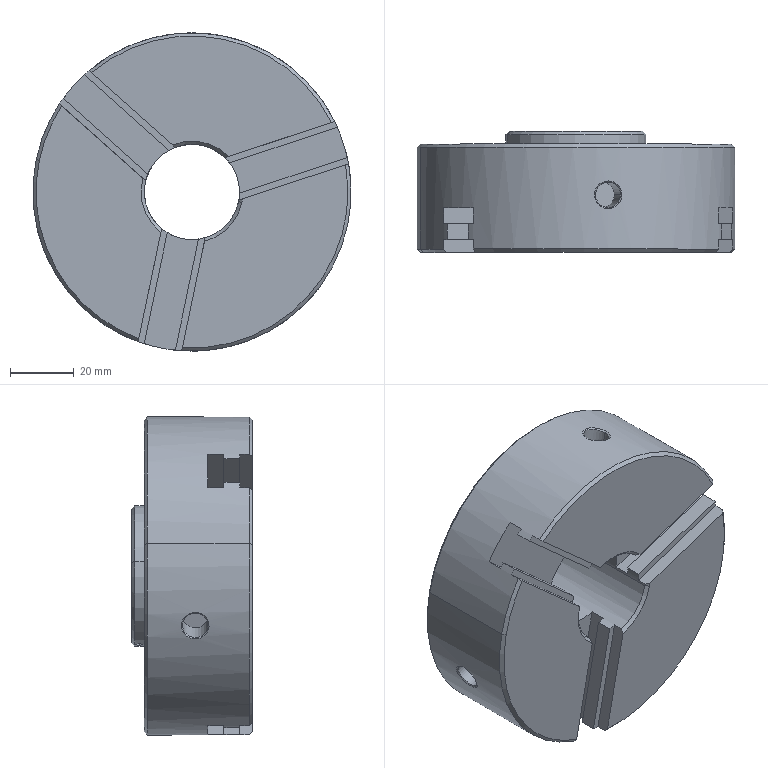Component | SolidWorks | HZ022-Three-JawChuck-1 | 1 solid | 80 faces | volume 224975 mm3 | plane 45 | cone 15 | cylinder 14 | spline 6 | commonest cylinder face diameters 8 x6 2 x2 44 x2 30 x2 100 x2